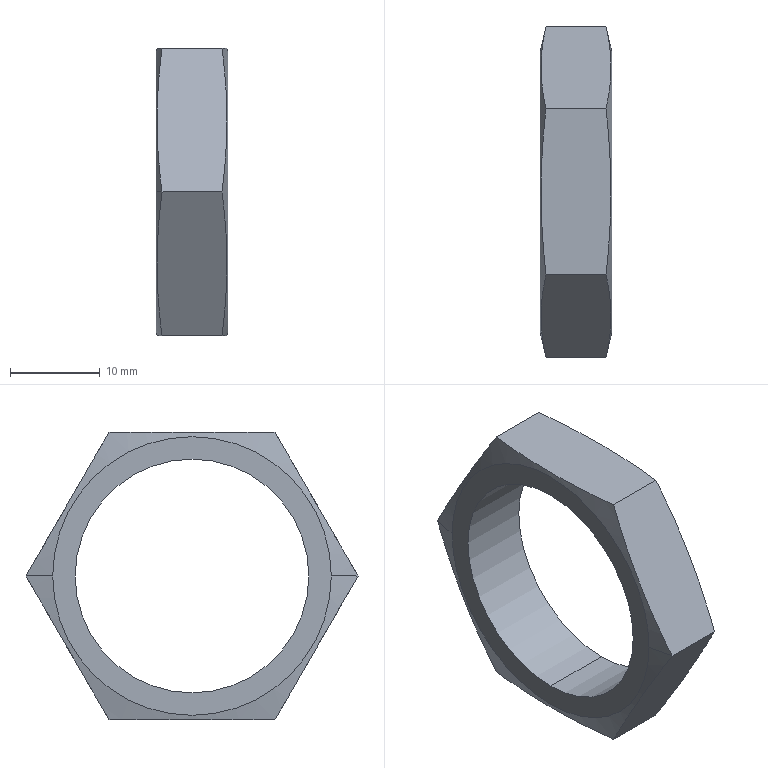Component | SolidWorks | RMS32X800_0-1_RMS32X50_Nut-1 | 1 solid | 14 faces | box 8 x 36.95 x 32 mm | volume 2796 mm3 | plane 8 | cone 4 | cylinder 2 | commonest cylinder face diameters 26 x2
STEP:
#1=COLOUR_RGB('',0.7922,0.8196,0.9333);
#2=FILL_AREA_STYLE_COLOUR('',#1);
#3=FILL_AREA_STYLE('',(#2));
#4=SURFACE_STYLE_FILL_AREA(#3);
#5=SURFACE_SIDE_STYLE('',(#4));
#6=SURFACE_STYLE_USAGE(.BOTH.,#5);
#7=PRESENTATION_STYLE_ASSIGNMENT((#6));
#8=CARTESIAN_POINT('',(-18.614,0.563,-15.472));
#9=VERTEX_POINT('',#8);
#10=CARTESIAN_POINT('',(-18.614,0.563,-14.449));
#11=VERTEX_POINT('',#10);
#12=CARTESIAN_POINT('',(-18.614,0.563,-14.961));
#13=DIRECTION('',(1.,0.,0.));
#14=DIRECTION('',(0.,0.,-1.));
#15=AXIS2_PLACEMENT_3D('',#12,#13,#14);
#16=CIRCLE('',#15,0.5118);
#17=EDGE_CURVE('',#9,#11,#16,.T.);
#18=ORIENTED_EDGE('',*,*,#17,.F.);
#19=CARTESIAN_POINT('',(-18.299,0.563,-15.472));
#20=VERTEX_POINT('',#19);
#21=CARTESIAN_POINT('',(-19.598,0.563,-15.472));
#22=DIRECTION('',(1.,0.,0.));
#23=VECTOR('',#22,39.37);
#24=LINE('',#21,#23);
#25=EDGE_CURVE('',#9,#20,#24,.T.);
#26=ORIENTED_EDGE('',*,*,#25,.T.);
#27=CARTESIAN_POINT('',(-18.299,0.563,-14.449));
#28=VERTEX_POINT('',#27);
#29=CARTESIAN_POINT('',(-18.299,0.563,-14.961));
#30=DIRECTION('',(-1.,-0.,-0.));
#31=DIRECTION('',(0.,0.,1.));
#32=AXIS2_PLACEMENT_3D('',#29,#30,#31);
#33=CIRCLE('',#32,0.5118);
#34=EDGE_CURVE('',#28,#20,#33,.T.);
#35=ORIENTED_EDGE('',*,*,#34,.F.);
#36=CARTESIAN_POINT('',(-19.598,0.563,-14.449));
#37=DIRECTION('',(1.,0.,0.));
#38=VECTOR('',#37,39.37);
#39=LINE('',#36,#38);
#40=EDGE_CURVE('',#11,#28,#39,.T.);
#41=ORIENTED_EDGE('',*,*,#40,.F.);
#42=EDGE_LOOP('',(#18,#26,#35,#41));
#43=FACE_OUTER_BOUND('',#42,.T.);
#44=CARTESIAN_POINT('',(-19.598,0.563,-14.961));
#45=DIRECTION('',(1.,0.,0.));
#46=DIRECTION('',(0.,0.,1.));
#47=AXIS2_PLACEMENT_3D('',#44,#45,#46);
#48=CYLINDRICAL_SURFACE('',#47,0.5118);
#49=ADVANCED_FACE('',(#43),#48,.F.);
#50=CARTESIAN_POINT('',(-18.299,0.563,-14.35));
#51=VERTEX_POINT('',#50);
#52=CARTESIAN_POINT('',(-18.299,0.563,-15.571));
#53=VERTEX_POINT('',#52);
#54=CARTESIAN_POINT('',(-18.299,0.563,-14.961));
#55=DIRECTION('',(1.,0.,0.));
#56=DIRECTION('',(0.,0.,-1.));
#57=AXIS2_PLACEMENT_3D('',#54,#55,#56);
#58=CIRCLE('',#57,0.6102);
#59=EDGE_CURVE('',#51,#53,#58,.T.);
#60=ORIENTED_EDGE('',*,*,#59,.F.);
#61=CARTESIAN_POINT('',(-18.303,0.563,-14.331));
#62=VERTEX_POINT('',#61);
#63=CARTESIAN_POINT('',(-18.325,0.563,-14.233));
#64=DIRECTION('',(-0.2176,-0.,0.976));
#65=VECTOR('',#64,39.37);
#66=LINE('',#63,#65);
#67=EDGE_CURVE('',#51,#62,#66,.T.);
#68=ORIENTED_EDGE('',*,*,#67,.T.);
#69=CARTESIAN_POINT('',(-18.325,0.1994,-14.331));
#70=VERTEX_POINT('',#69);
#71=CARTESIAN_POINT('',(-18.303,0.563,-14.331));
#72=CARTESIAN_POINT('',(-18.303,0.5024,-14.331));
#73=CARTESIAN_POINT('',(-18.305,0.4418,-14.331));
#74=CARTESIAN_POINT('',(-18.313,0.3206,-14.331));
#75=CARTESIAN_POINT('',(-18.318,0.26,-14.331));
#76=CARTESIAN_POINT('',(-18.325,0.1994,-14.331));
#77=B_SPLINE_CURVE_WITH_KNOTS('',3,(#71,#72,#73,#74,#75,#76),.UNSPECIFIED.,.F.,.F.,(4,2,4),(0.009238,0.01386,0.01848),.UNSPECIFIED.);
#78=EDGE_CURVE('',#62,#70,#77,.T.);
#79=ORIENTED_EDGE('',*,*,#78,.T.);
#80=CARTESIAN_POINT('',(-18.325,-0.1643,-14.961));
#81=VERTEX_POINT('',#80);
#82=CARTESIAN_POINT('',(-18.325,0.1994,-14.331));
#83=CARTESIAN_POINT('',(-18.318,0.169,-14.383));
#84=CARTESIAN_POINT('',(-18.313,0.1387,-14.436));
#85=CARTESIAN_POINT('',(-18.305,0.07813,-14.541));
#86=CARTESIAN_POINT('',(-18.301,0.01751,-14.646));
#87=CARTESIAN_POINT('',(-18.305,-0.0431,-14.751));
#88=CARTESIAN_POINT('',(-18.313,-0.1037,-14.856));
#89=CARTESIAN_POINT('',(-18.318,-0.134,-14.908));
#90=CARTESIAN_POINT('',(-18.325,-0.1643,-14.961));
#91=B_SPLINE_CURVE_WITH_KNOTS('',3,(#82,#83,#84,#85,#86,#87,#88,#89,#90),.UNSPECIFIED.,.F.,.F.,(4,2,1,2,4),(0.,0.004619,0.009238,0.01386,0.01848),.UNSPECIFIED.);
#92=EDGE_CURVE('',#70,#81,#91,.T.);
#93=ORIENTED_EDGE('',*,*,#92,.T.);
#94=CARTESIAN_POINT('',(-18.325,0.1994,-15.591));
#95=VERTEX_POINT('',#94);
#96=CARTESIAN_POINT('',(-18.325,-0.1643,-14.961));
#97=CARTESIAN_POINT('',(-18.318,-0.134,-15.013));
#98=CARTESIAN_POINT('',(-18.313,-0.1037,-15.066));
#99=CARTESIAN_POINT('',(-18.305,-0.0431,-15.171));
#100=CARTESIAN_POINT('',(-18.301,0.01751,-15.276));
#101=CARTESIAN_POINT('',(-18.305,0.07813,-15.381));
#102=CARTESIAN_POINT('',(-18.313,0.1387,-15.486));
#103=CARTESIAN_POINT('',(-18.318,0.169,-15.538));
#104=CARTESIAN_POINT('',(-18.325,0.1994,-15.591));
#105=B_SPLINE_CURVE_WITH_KNOTS('',3,(#96,#97,#98,#99,#100,#101,#102,#103,#104),.UNSPECIFIED.,.F.,.F.,(4,2,1,2,4),(0.,0.004619,0.009238,0.01386,0.01848),.UNSPECIFIED.);
#106=EDGE_CURVE('',#81,#95,#105,.T.);
#107=ORIENTED_EDGE('',*,*,#106,.T.);
#108=CARTESIAN_POINT('',(-18.303,0.563,-15.591));
#109=VERTEX_POINT('',#108);
#110=CARTESIAN_POINT('',(-18.325,0.1994,-15.591));
#111=CARTESIAN_POINT('',(-18.318,0.26,-15.591));
#112=CARTESIAN_POINT('',(-18.313,0.3206,-15.591));
#113=CARTESIAN_POINT('',(-18.305,0.4418,-15.591));
#114=CARTESIAN_POINT('',(-18.303,0.5024,-15.591));
#115=CARTESIAN_POINT('',(-18.303,0.563,-15.591));
#116=B_SPLINE_CURVE_WITH_KNOTS('',3,(#110,#111,#112,#113,#114,#115),.UNSPECIFIED.,.F.,.F.,(4,2,4),(0.,0.004619,0.009238),.UNSPECIFIED.);
#117=EDGE_CURVE('',#95,#109,#116,.T.);
#118=ORIENTED_EDGE('',*,*,#117,.T.);
#119=CARTESIAN_POINT('',(-18.325,0.563,-15.689));
#120=DIRECTION('',(-0.2176,0.,-0.976));
#121=VECTOR('',#120,39.37);
#122=LINE('',#119,#121);
#123=EDGE_CURVE('',#53,#109,#122,.T.);
#124=ORIENTED_EDGE('',*,*,#123,.F.);
#125=EDGE_LOOP('',(#60,#68,#79,#93,#107,#118,#124));
#126=FACE_OUTER_BOUND('',#125,.T.);
#127=CARTESIAN_POINT('',(-18.325,0.563,-14.961));
#128=DIRECTION('',(-1.,-0.,-0.));
#129=DIRECTION('',(0.,0.,-1.));
#130=AXIS2_PLACEMENT_3D('',#127,#128,#129);
#131=CONICAL_SURFACE('',#130,0.7281,1.351);
#132=ADVANCED_FACE('',(#126),#131,.T.);
#133=CARTESIAN_POINT('',(-18.614,1.173,-14.961));
#134=VERTEX_POINT('',#133);
#135=CARTESIAN_POINT('',(-18.614,-0.0472,-14.961));
#136=VERTEX_POINT('',#135);
#137=CARTESIAN_POINT('',(-18.614,0.563,-14.961));
#138=DIRECTION('',(-1.,-0.,-0.));
#139=DIRECTION('',(0.,-1.,0.));
#140=AXIS2_PLACEMENT_3D('',#137,#138,#139);
#141=CIRCLE('',#140,0.6102);
#142=EDGE_CURVE('',#134,#136,#141,.T.);
#143=ORIENTED_EDGE('',*,*,#142,.F.);
#144=CARTESIAN_POINT('',(-18.588,1.29,-14.961));
#145=VERTEX_POINT('',#144);
#146=CARTESIAN_POINT('',(-18.588,1.291,-14.961));
#147=DIRECTION('',(0.2176,0.976,-0.));
#148=VECTOR('',#147,39.37);
#149=LINE('',#146,#148);
#150=EDGE_CURVE('',#134,#145,#149,.T.);
#151=ORIENTED_EDGE('',*,*,#150,.T.);
#152=CARTESIAN_POINT('',(-18.588,0.9267,-15.591));
#153=VERTEX_POINT('',#152);
#154=CARTESIAN_POINT('',(-18.588,1.29,-14.961));
#155=CARTESIAN_POINT('',(-18.594,1.26,-15.013));
#156=CARTESIAN_POINT('',(-18.6,1.23,-15.066));
#157=CARTESIAN_POINT('',(-18.607,1.169,-15.171));
#158=CARTESIAN_POINT('',(-18.611,1.109,-15.276));
#159=CARTESIAN_POINT('',(-18.607,1.048,-15.381));
#160=CARTESIAN_POINT('',(-18.6,0.9873,-15.486));
#161=CARTESIAN_POINT('',(-18.594,0.957,-15.538));
#162=CARTESIAN_POINT('',(-18.588,0.9267,-15.591));
#163=B_SPLINE_CURVE_WITH_KNOTS('',3,(#154,#155,#156,#157,#158,#159,#160,#161,#162),.UNSPECIFIED.,.F.,.F.,(4,2,1,2,4),(0.,0.004619,0.009238,0.01386,0.01848),.UNSPECIFIED.);
#164=EDGE_CURVE('',#145,#153,#163,.T.);
#165=ORIENTED_EDGE('',*,*,#164,.T.);
#166=CARTESIAN_POINT('',(-18.588,0.1994,-15.591));
#167=VERTEX_POINT('',#166);
#168=CARTESIAN_POINT('',(-18.588,0.9267,-15.591));
#169=CARTESIAN_POINT('',(-18.594,0.8661,-15.591));
#170=CARTESIAN_POINT('',(-18.6,0.8055,-15.591));
#171=CARTESIAN_POINT('',(-18.607,0.6843,-15.591));
#172=CARTESIAN_POINT('',(-18.611,0.563,-15.591));
#173=CARTESIAN_POINT('',(-18.607,0.4418,-15.591));
#174=CARTESIAN_POINT('',(-18.6,0.3206,-15.591));
#175=CARTESIAN_POINT('',(-18.594,0.26,-15.591));
#176=CARTESIAN_POINT('',(-18.588,0.1994,-15.591));
#177=B_SPLINE_CURVE_WITH_KNOTS('',3,(#168,#169,#170,#171,#172,#173,#174,#175,#176),.UNSPECIFIED.,.F.,.F.,(4,2,1,2,4),(0.,0.004619,0.009238,0.01386,0.01848),.UNSPECIFIED.);
#178=EDGE_CURVE('',#153,#167,#177,.T.);
#179=ORIENTED_EDGE('',*,*,#178,.T.);
#180=CARTESIAN_POINT('',(-18.588,-0.1643,-14.961));
#181=VERTEX_POINT('',#180);
#182=CARTESIAN_POINT('',(-18.588,0.1994,-15.591));
#183=CARTESIAN_POINT('',(-18.594,0.169,-15.538));
#184=CARTESIAN_POINT('',(-18.6,0.1387,-15.486));
#185=CARTESIAN_POINT('',(-18.607,0.07813,-15.381));
#186=CARTESIAN_POINT('',(-18.611,0.01751,-15.276));
#187=CARTESIAN_POINT('',(-18.607,-0.0431,-15.171));
#188=CARTESIAN_POINT('',(-18.6,-0.1037,-15.066));
#189=CARTESIAN_POINT('',(-18.594,-0.134,-15.013));
#190=CARTESIAN_POINT('',(-18.588,-0.1643,-14.961));
#191=B_SPLINE_CURVE_WITH_KNOTS('',3,(#182,#183,#184,#185,#186,#187,#188,#189,#190),.UNSPECIFIED.,.F.,.F.,(4,2,1,2,4),(0.,0.004619,0.009238,0.01386,0.01848),.UNSPECIFIED.);
#192=EDGE_CURVE('',#167,#181,#191,.T.);
#193=ORIENTED_EDGE('',*,*,#192,.T.);
#194=CARTESIAN_POINT('',(-18.588,-0.165,-14.961));
#195=DIRECTION('',(0.2176,-0.976,-0.));
#196=VECTOR('',#195,39.37);
#197=LINE('',#194,#196);
#198=EDGE_CURVE('',#136,#181,#197,.T.);
#199=ORIENTED_EDGE('',*,*,#198,.F.);
#200=EDGE_LOOP('',(#143,#151,#165,#179,#193,#199));
#201=FACE_OUTER_BOUND('',#200,.T.);
#202=CARTESIAN_POINT('',(-18.588,0.563,-14.961));
#203=DIRECTION('',(1.,0.,0.));
#204=DIRECTION('',(0.,-1.,0.));
#205=AXIS2_PLACEMENT_3D('',#202,#203,#204);
#206=CONICAL_SURFACE('',#205,0.7281,1.351);
#207=ADVANCED_FACE('',(#201),#206,.T.);
#208=CARTESIAN_POINT('',(-18.299,0.563,-14.961));
#209=DIRECTION('',(1.,0.,0.));
#210=DIRECTION('',(0.,0.,-1.));
#211=AXIS2_PLACEMENT_3D('',#208,#209,#210);
#212=CIRCLE('',#211,0.6102);
#213=EDGE_CURVE('',#53,#51,#212,.T.);
#214=ORIENTED_EDGE('',*,*,#213,.T.);
#215=ORIENTED_EDGE('',*,*,#59,.T.);
#216=EDGE_LOOP('',(#214,#215));
#217=FACE_OUTER_BOUND('',#216,.T.);
#218=ORIENTED_EDGE('',*,*,#34,.T.);
#219=CARTESIAN_POINT('',(-18.299,0.563,-14.961));
#220=DIRECTION('',(-1.,-0.,-0.));
#221=DIRECTION('',(0.,0.,1.));
#222=AXIS2_PLACEMENT_3D('',#219,#220,#221);
#223=CIRCLE('',#222,0.5118);
#224=EDGE_CURVE('',#20,#28,#223,.T.);
#225=ORIENTED_EDGE('',*,*,#224,.T.);
#226=EDGE_LOOP('',(#218,#225));
#227=FACE_BOUND('',#226,.T.);
#228=CARTESIAN_POINT('',(-18.299,1.173,-14.961));
#229=DIRECTION('',(1.,0.,0.));
#230=DIRECTION('',(-0.,-0.,1.));
#231=AXIS2_PLACEMENT_3D('',#228,#229,#230);
#232=PLANE('',#231);
#233=ADVANCED_FACE('',(#217,#227),#232,.T.);
#234=CARTESIAN_POINT('',(-18.614,0.563,-14.961));
#235=DIRECTION('',(1.,0.,0.));
#236=DIRECTION('',(0.,0.,-1.));
#237=AXIS2_PLACEMENT_3D('',#234,#235,#236);
#238=CIRCLE('',#237,0.5118);
#239=EDGE_CURVE('',#11,#9,#238,.T.);
#240=ORIENTED_EDGE('',*,*,#239,.T.);
#241=ORIENTED_EDGE('',*,*,#17,.T.);
#242=EDGE_LOOP('',(#240,#241));
#243=FACE_BOUND('',#242,.T.);
#244=CARTESIAN_POINT('',(-18.614,0.563,-14.961));
#245=DIRECTION('',(-1.,-0.,-0.));
#246=DIRECTION('',(0.,-1.,0.));
#247=AXIS2_PLACEMENT_3D('',#244,#245,#246);
#248=CIRCLE('',#247,0.6102);
#249=EDGE_CURVE('',#136,#134,#248,.T.);
#250=ORIENTED_EDGE('',*,*,#249,.T.);
#251=ORIENTED_EDGE('',*,*,#142,.T.);
#252=EDGE_LOOP('',(#250,#251));
#253=FACE_OUTER_BOUND('',#252,.T.);
#254=CARTESIAN_POINT('',(-18.614,1.075,-14.961));
#255=DIRECTION('',(-1.,-0.,-0.));
#256=DIRECTION('',(0.,0.,-1.));
#257=AXIS2_PLACEMENT_3D('',#254,#255,#256);
#258=PLANE('',#257);
#259=ADVANCED_FACE('',(#243,#253),#258,.T.);
#260=ORIENTED_EDGE('',*,*,#67,.F.);
#261=ORIENTED_EDGE('',*,*,#213,.F.);
#262=ORIENTED_EDGE('',*,*,#123,.T.);
#263=CARTESIAN_POINT('',(-18.325,0.9267,-15.591));
#264=VERTEX_POINT('',#263);
#265=CARTESIAN_POINT('',(-18.303,0.563,-15.591));
#266=CARTESIAN_POINT('',(-18.303,0.6237,-15.591));
#267=CARTESIAN_POINT('',(-18.305,0.6843,-15.591));
#268=CARTESIAN_POINT('',(-18.313,0.8055,-15.591));
#269=CARTESIAN_POINT('',(-18.318,0.8661,-15.591));
#270=CARTESIAN_POINT('',(-18.325,0.9267,-15.591));
#271=B_SPLINE_CURVE_WITH_KNOTS('',3,(#265,#266,#267,#268,#269,#270),.UNSPECIFIED.,.F.,.F.,(4,2,4),(0.009238,0.01386,0.01848),.UNSPECIFIED.);
#272=EDGE_CURVE('',#109,#264,#271,.T.);
#273=ORIENTED_EDGE('',*,*,#272,.T.);
#274=CARTESIAN_POINT('',(-18.325,1.29,-14.961));
#275=VERTEX_POINT('',#274);
#276=CARTESIAN_POINT('',(-18.325,0.9267,-15.591));
#277=CARTESIAN_POINT('',(-18.318,0.957,-15.538));
#278=CARTESIAN_POINT('',(-18.313,0.9873,-15.486));
#279=CARTESIAN_POINT('',(-18.305,1.048,-15.381));
#280=CARTESIAN_POINT('',(-18.301,1.109,-15.276));
#281=CARTESIAN_POINT('',(-18.305,1.169,-15.171));
#282=CARTESIAN_POINT('',(-18.313,1.23,-15.066));
#283=CARTESIAN_POINT('',(-18.318,1.26,-15.013));
#284=CARTESIAN_POINT('',(-18.325,1.29,-14.961));
#285=B_SPLINE_CURVE_WITH_KNOTS('',3,(#276,#277,#278,#279,#280,#281,#282,#283,#284),.UNSPECIFIED.,.F.,.F.,(4,2,1,2,4),(0.,0.004619,0.009238,0.01386,0.01848),.UNSPECIFIED.);
#286=EDGE_CURVE('',#264,#275,#285,.T.);
#287=ORIENTED_EDGE('',*,*,#286,.T.);
#288=CARTESIAN_POINT('',(-18.325,0.9267,-14.331));
#289=VERTEX_POINT('',#288);
#290=CARTESIAN_POINT('',(-18.325,1.29,-14.961));
#291=CARTESIAN_POINT('',(-18.318,1.26,-14.908));
#292=CARTESIAN_POINT('',(-18.313,1.23,-14.856));
#293=CARTESIAN_POINT('',(-18.305,1.169,-14.751));
#294=CARTESIAN_POINT('',(-18.301,1.109,-14.646));
#295=CARTESIAN_POINT('',(-18.305,1.048,-14.541));
#296=CARTESIAN_POINT('',(-18.313,0.9873,-14.436));
#297=CARTESIAN_POINT('',(-18.318,0.957,-14.383));
#298=CARTESIAN_POINT('',(-18.325,0.9267,-14.331));
#299=B_SPLINE_CURVE_WITH_KNOTS('',3,(#290,#291,#292,#293,#294,#295,#296,#297,#298),.UNSPECIFIED.,.F.,.F.,(4,2,1,2,4),(0.,0.004619,0.009238,0.01386,0.01848),.UNSPECIFIED.);
#300=EDGE_CURVE('',#275,#289,#299,.T.);
#301=ORIENTED_EDGE('',*,*,#300,.T.);
#302=CARTESIAN_POINT('',(-18.325,0.9267,-14.331));
#303=CARTESIAN_POINT('',(-18.318,0.8661,-14.331));
#304=CARTESIAN_POINT('',(-18.313,0.8055,-14.331));
#305=CARTESIAN_POINT('',(-18.305,0.6843,-14.331));
#306=CARTESIAN_POINT('',(-18.303,0.6237,-14.331));
#307=CARTESIAN_POINT('',(-18.303,0.563,-14.331));
#308=B_SPLINE_CURVE_WITH_KNOTS('',3,(#302,#303,#304,#305,#306,#307),.UNSPECIFIED.,.F.,.F.,(4,2,4),(0.,0.004619,0.009238),.UNSPECIFIED.);
#309=EDGE_CURVE('',#289,#62,#308,.T.);
#310=ORIENTED_EDGE('',*,*,#309,.T.);
#311=EDGE_LOOP('',(#260,#261,#262,#273,#287,#301,#310));
#312=FACE_OUTER_BOUND('',#311,.T.);
#313=CARTESIAN_POINT('',(-18.325,0.563,-14.961));
#314=DIRECTION('',(-1.,-0.,-0.));
#315=DIRECTION('',(0.,0.,-1.));
#316=AXIS2_PLACEMENT_3D('',#313,#314,#315);
#317=CONICAL_SURFACE('',#316,0.7281,1.351);
#318=ADVANCED_FACE('',(#312),#317,.T.);
#319=ORIENTED_EDGE('',*,*,#150,.F.);
#320=ORIENTED_EDGE('',*,*,#249,.F.);
#321=ORIENTED_EDGE('',*,*,#198,.T.);
#322=CARTESIAN_POINT('',(-18.588,0.1994,-14.331));
#323=VERTEX_POINT('',#322);
#324=CARTESIAN_POINT('',(-18.588,-0.1643,-14.961));
#325=CARTESIAN_POINT('',(-18.594,-0.134,-14.908));
#326=CARTESIAN_POINT('',(-18.6,-0.1037,-14.856));
#327=CARTESIAN_POINT('',(-18.607,-0.0431,-14.751));
#328=CARTESIAN_POINT('',(-18.611,0.01751,-14.646));
#329=CARTESIAN_POINT('',(-18.607,0.07813,-14.541));
#330=CARTESIAN_POINT('',(-18.6,0.1387,-14.436));
#331=CARTESIAN_POINT('',(-18.594,0.169,-14.383));
#332=CARTESIAN_POINT('',(-18.588,0.1994,-14.331));
#333=B_SPLINE_CURVE_WITH_KNOTS('',3,(#324,#325,#326,#327,#328,#329,#330,#331,#332),.UNSPECIFIED.,.F.,.F.,(4,2,1,2,4),(0.,0.004619,0.009238,0.01386,0.01848),.UNSPECIFIED.);
#334=EDGE_CURVE('',#181,#323,#333,.T.);
#335=ORIENTED_EDGE('',*,*,#334,.T.);
#336=CARTESIAN_POINT('',(-18.588,0.9267,-14.331));
#337=VERTEX_POINT('',#336);
#338=CARTESIAN_POINT('',(-18.588,0.1994,-14.331));
#339=CARTESIAN_POINT('',(-18.594,0.26,-14.331));
#340=CARTESIAN_POINT('',(-18.6,0.3206,-14.331));
#341=CARTESIAN_POINT('',(-18.607,0.4418,-14.331));
#342=CARTESIAN_POINT('',(-18.611,0.563,-14.331));
#343=CARTESIAN_POINT('',(-18.607,0.6843,-14.331));
#344=CARTESIAN_POINT('',(-18.6,0.8055,-14.331));
#345=CARTESIAN_POINT('',(-18.594,0.8661,-14.331));
#346=CARTESIAN_POINT('',(-18.588,0.9267,-14.331));
#347=B_SPLINE_CURVE_WITH_KNOTS('',3,(#338,#339,#340,#341,#342,#343,#344,#345,#346),.UNSPECIFIED.,.F.,.F.,(4,2,1,2,4),(0.,0.004619,0.009238,0.01386,0.01848),.UNSPECIFIED.);
#348=EDGE_CURVE('',#323,#337,#347,.T.);
#349=ORIENTED_EDGE('',*,*,#348,.T.);
#350=CARTESIAN_POINT('',(-18.588,0.9267,-14.331));
#351=CARTESIAN_POINT('',(-18.594,0.957,-14.383));
#352=CARTESIAN_POINT('',(-18.6,0.9873,-14.436));
#353=CARTESIAN_POINT('',(-18.607,1.048,-14.541));
#354=CARTESIAN_POINT('',(-18.611,1.109,-14.646));
#355=CARTESIAN_POINT('',(-18.607,1.169,-14.751));
#356=CARTESIAN_POINT('',(-18.6,1.23,-14.856));
#357=CARTESIAN_POINT('',(-18.594,1.26,-14.908));
#358=CARTESIAN_POINT('',(-18.588,1.29,-14.961));
#359=B_SPLINE_CURVE_WITH_KNOTS('',3,(#350,#351,#352,#353,#354,#355,#356,#357,#358),.UNSPECIFIED.,.F.,.F.,(4,2,1,2,4),(0.,0.004619,0.009238,0.01386,0.01848),.UNSPECIFIED.);
#360=EDGE_CURVE('',#337,#145,#359,.T.);
#361=ORIENTED_EDGE('',*,*,#360,.T.);
#362=EDGE_LOOP('',(#319,#320,#321,#335,#349,#361));
#363=FACE_OUTER_BOUND('',#362,.T.);
#364=CARTESIAN_POINT('',(-18.588,0.563,-14.961));
#365=DIRECTION('',(1.,0.,0.));
#366=DIRECTION('',(0.,-1.,0.));
#367=AXIS2_PLACEMENT_3D('',#364,#365,#366);
#368=CONICAL_SURFACE('',#367,0.7281,1.351);
#369=ADVANCED_FACE('',(#363),#368,.T.);
#370=CARTESIAN_POINT('',(-18.299,0.1994,-15.591));
#371=DIRECTION('',(-1.,-0.,-0.));
#372=VECTOR('',#371,39.37);
#373=LINE('',#370,#372);
#374=EDGE_CURVE('',#95,#167,#373,.T.);
#375=ORIENTED_EDGE('',*,*,#374,.F.);
#376=ORIENTED_EDGE('',*,*,#106,.F.);
#377=CARTESIAN_POINT('',(-18.299,-0.1643,-14.961));
#378=DIRECTION('',(1.,0.,0.));
#379=VECTOR('',#378,39.37);
#380=LINE('',#377,#379);
#381=EDGE_CURVE('',#181,#81,#380,.T.);
#382=ORIENTED_EDGE('',*,*,#381,.F.);
#383=ORIENTED_EDGE('',*,*,#192,.F.);
#384=EDGE_LOOP('',(#375,#376,#382,#383));
#385=FACE_OUTER_BOUND('',#384,.T.);
#386=CARTESIAN_POINT('',(-18.299,-0.1643,-14.961));
#387=DIRECTION('',(-0.,0.866,0.5));
#388=DIRECTION('',(-0.,-0.5,0.866));
#389=AXIS2_PLACEMENT_3D('',#386,#387,#388);
#390=PLANE('',#389);
#391=ADVANCED_FACE('',(#385),#390,.F.);
#392=ORIENTED_EDGE('',*,*,#381,.T.);
#393=ORIENTED_EDGE('',*,*,#92,.F.);
#394=CARTESIAN_POINT('',(-18.299,0.1994,-14.331));
#395=DIRECTION('',(1.,0.,0.));
#396=VECTOR('',#395,39.37);
#397=LINE('',#394,#396);
#398=EDGE_CURVE('',#323,#70,#397,.T.);
#399=ORIENTED_EDGE('',*,*,#398,.F.);
#400=ORIENTED_EDGE('',*,*,#334,.F.);
#401=EDGE_LOOP('',(#392,#393,#399,#400));
#402=FACE_OUTER_BOUND('',#401,.T.);
#403=CARTESIAN_POINT('',(-18.299,0.1994,-14.331));
#404=DIRECTION('',(-0.,0.866,-0.5));
#405=DIRECTION('',(-0.,0.5,0.866));
#406=AXIS2_PLACEMENT_3D('',#403,#404,#405);
#407=PLANE('',#406);
#408=ADVANCED_FACE('',(#402),#407,.F.);
#409=ORIENTED_EDGE('',*,*,#398,.T.);
#410=ORIENTED_EDGE('',*,*,#78,.F.);
#411=ORIENTED_EDGE('',*,*,#309,.F.);
#412=CARTESIAN_POINT('',(-18.299,0.9267,-14.331));
#413=DIRECTION('',(1.,0.,0.));
#414=VECTOR('',#413,39.37);
#415=LINE('',#412,#414);
#416=EDGE_CURVE('',#337,#289,#415,.T.);
#417=ORIENTED_EDGE('',*,*,#416,.F.);
#418=ORIENTED_EDGE('',*,*,#348,.F.);
#419=EDGE_LOOP('',(#409,#410,#411,#417,#418));
#420=FACE_OUTER_BOUND('',#419,.T.);
#421=CARTESIAN_POINT('',(-18.299,0.9267,-14.331));
#422=DIRECTION('',(0.,0.,-1.));
#423=DIRECTION('',(1.,0.,0.));
#424=AXIS2_PLACEMENT_3D('',#421,#422,#423);
#425=PLANE('',#424);
#426=ADVANCED_FACE('',(#420),#425,.F.);
#427=ORIENTED_EDGE('',*,*,#416,.T.);
#428=ORIENTED_EDGE('',*,*,#300,.F.);
#429=CARTESIAN_POINT('',(-18.299,1.29,-14.961));
#430=DIRECTION('',(1.,0.,0.));
#431=VECTOR('',#430,39.37);
#432=LINE('',#429,#431);
#433=EDGE_CURVE('',#145,#275,#432,.T.);
#434=ORIENTED_EDGE('',*,*,#433,.F.);
#435=ORIENTED_EDGE('',*,*,#360,.F.);
#436=EDGE_LOOP('',(#427,#428,#434,#435));
#437=FACE_OUTER_BOUND('',#436,.T.);
#438=CARTESIAN_POINT('',(-18.299,1.29,-14.961));
#439=DIRECTION('',(0.,-0.866,-0.5));
#440=DIRECTION('',(0.,0.5,-0.866));
#441=AXIS2_PLACEMENT_3D('',#438,#439,#440);
#442=PLANE('',#441);
#443=ADVANCED_FACE('',(#437),#442,.F.);
#444=ORIENTED_EDGE('',*,*,#433,.T.);
#445=ORIENTED_EDGE('',*,*,#286,.F.);
#446=CARTESIAN_POINT('',(-18.299,0.9267,-15.591));
#447=DIRECTION('',(1.,0.,0.));
#448=VECTOR('',#447,39.37);
#449=LINE('',#446,#448);
#450=EDGE_CURVE('',#153,#264,#449,.T.);
#451=ORIENTED_EDGE('',*,*,#450,.F.);
#452=ORIENTED_EDGE('',*,*,#164,.F.);
#453=EDGE_LOOP('',(#444,#445,#451,#452));
#454=FACE_OUTER_BOUND('',#453,.T.);
#455=CARTESIAN_POINT('',(-18.299,0.9267,-15.591));
#456=DIRECTION('',(0.,-0.866,0.5));
#457=DIRECTION('',(0.,-0.5,-0.866));
#458=AXIS2_PLACEMENT_3D('',#455,#456,#457);
#459=PLANE('',#458);
#460=ADVANCED_FACE('',(#454),#459,.F.);
#461=ORIENTED_EDGE('',*,*,#450,.T.);
#462=ORIENTED_EDGE('',*,*,#272,.F.);
#463=ORIENTED_EDGE('',*,*,#117,.F.);
#464=ORIENTED_EDGE('',*,*,#374,.T.);
#465=ORIENTED_EDGE('',*,*,#178,.F.);
#466=EDGE_LOOP('',(#461,#462,#463,#464,#465));
#467=FACE_OUTER_BOUND('',#466,.T.);
#468=CARTESIAN_POINT('',(-18.299,0.1994,-15.591));
#469=DIRECTION('',(-0.,-0.,1.));
#470=DIRECTION('',(-1.,-0.,-0.));
#471=AXIS2_PLACEMENT_3D('',#468,#469,#470);
#472=PLANE('',#471);
#473=ADVANCED_FACE('',(#467),#472,.F.);
#474=ORIENTED_EDGE('',*,*,#25,.F.);
#475=ORIENTED_EDGE('',*,*,#239,.F.);
#476=ORIENTED_EDGE('',*,*,#40,.T.);
#477=ORIENTED_EDGE('',*,*,#224,.F.);
#478=EDGE_LOOP('',(#474,#475,#476,#477));
#479=FACE_OUTER_BOUND('',#478,.T.);
#480=CARTESIAN_POINT('',(-19.598,0.563,-14.961));
#481=DIRECTION('',(1.,0.,0.));
#482=DIRECTION('',(0.,0.,1.));
#483=AXIS2_PLACEMENT_3D('',#480,#481,#482);
#484=CYLINDRICAL_SURFACE('',#483,0.5118);
#485=ADVANCED_FACE('',(#479),#484,.F.);
#486=CLOSED_SHELL('',(#49,#132,#207,#233,#259,#318,#369,#391,#408,#426,#443,#460,#473,#485));
#487=MANIFOLD_SOLID_BREP('',#486);
#488=STYLED_ITEM('',(#7),#487);
#489=PRESENTATION_LAYER_ASSIGNMENT('','',(#488));
#490=CARTESIAN_POINT('',(0.,0.,0.));
#491=DIRECTION('',(0.,0.,1.));
#492=DIRECTION('',(1.,0.,0.));
#493=AXIS2_PLACEMENT_3D('',#490,#491,#492);
#494=(LENGTH_UNIT()NAMED_UNIT(*)SI_UNIT($,.METRE.));
#495=LENGTH_MEASURE_WITH_UNIT(LENGTH_MEASURE(0.0254),#494);
#496=DIMENSIONAL_EXPONENTS(1.,0.,0.,0.,0.,0.,0.);
#497=(CONVERSION_BASED_UNIT('',#495)LENGTH_UNIT()NAMED_UNIT(#496));
#498=UNCERTAINTY_MEASURE_WITH_UNIT(LENGTH_MEASURE(0.00001),#497,'','');
#499=(NAMED_UNIT(*)PLANE_ANGLE_UNIT()SI_UNIT($,.RADIAN.));
#500=(NAMED_UNIT(*)SI_UNIT($,.STERADIAN.)SOLID_ANGLE_UNIT());
#501=(GEOMETRIC_REPRESENTATION_CONTEXT(3)GLOBAL_UNCERTAINTY_ASSIGNED_CONTEXT((#498))GLOBAL_UNIT_ASSIGNED_CONTEXT((#497,#499,#500))REPRESENTATION_CONTEXT('',''));
#502=ADVANCED_BREP_SHAPE_REPRESENTATION('',(#487,#493),#501);
#503=(LENGTH_UNIT()NAMED_UNIT(*)SI_UNIT($,.METRE.));
#504=LENGTH_MEASURE_WITH_UNIT(LENGTH_MEASURE(0.0254),#503);
#505=DIMENSIONAL_EXPONENTS(1.,0.,0.,0.,0.,0.,0.);
#506=(CONVERSION_BASED_UNIT('',#504)LENGTH_UNIT()NAMED_UNIT(#505));
#507=UNCERTAINTY_MEASURE_WITH_UNIT(LENGTH_MEASURE(0.00001),#506,'','');
#508=(NAMED_UNIT(*)PLANE_ANGLE_UNIT()SI_UNIT($,.RADIAN.));
#509=(NAMED_UNIT(*)SI_UNIT($,.STERADIAN.)SOLID_ANGLE_UNIT());
#510=(GEOMETRIC_REPRESENTATION_CONTEXT(3)GLOBAL_UNCERTAINTY_ASSIGNED_CONTEXT((#507))GLOBAL_UNIT_ASSIGNED_CONTEXT((#506,#508,#509))REPRESENTATION_CONTEXT('',''));
#511=MECHANICAL_DESIGN_GEOMETRIC_PRESENTATION_REPRESENTATION('',(#488),#510);